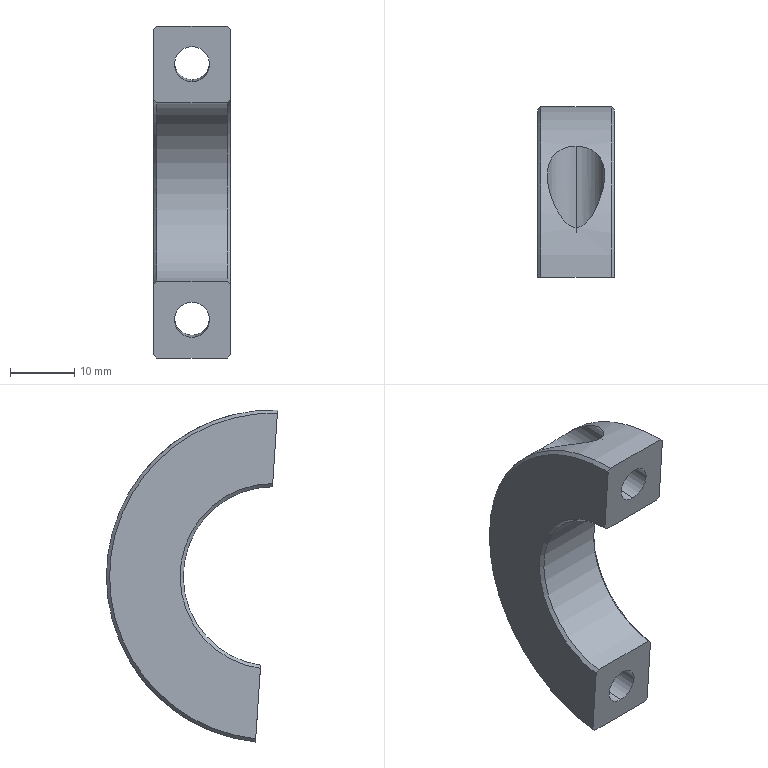Component | SolidWorks | TC020.05-07-1 | 1 solid | 20 faces | box 12 x 26.73 x 51.86 mm | volume 7193 mm3 | cylinder 10 | plane 6 | cone 4 | commonest cylinder face diameters 5.5 x4 9 x4 28 x1 52 x1 | material Q235A
build123d program:
from build123d import *

# Parameters (mm, degrees)
SKETCH1_W          = 12
SKETCH1_H          = 12
SKETCH2_W          = 52
SKETCH2_H          = 2
CUT_EXTRUDE1_DEPTH = 39.678
CHAMFER1_SIZE      = 0.5


with BuildPart() as part:
    # Sketch1 → Revolve1 (revolve)
    with BuildSketch(Plane.XY, mode=Mode.PRIVATE) as revolve1_sk:
        with Locations((0, 20)):
            Rectangle(SKETCH1_W, SKETCH1_H)
    revolve(revolve1_sk.sketch.rotate(Axis((0, 0, 0), (1, 0, 0)), 90), axis=Axis((0, 0, 0), (1, 0, 0)))

    # Sketch2 → Cut-Extrude1 (cut, through all)
    with BuildSketch(Plane(origin=(6, 0, 0), x_dir=(0, 0, -1), z_dir=(1, 0, 0))):
        Rectangle(SKETCH2_W, SKETCH2_H)
    extrude(amount=-CUT_EXTRUDE1_DEPTH, mode=Mode.SUBTRACT)


with BuildPart() as cut_extrude1_kept_piece:
    # of the separate pieces the step leaves, the one the design keeps (cut_extrude1_pieces_kept)
    add(part.part.solids().sort_by_distance((-6, 1, -13.964))[0])

    # Sketch5 → Cut-Revolve1 (revolve, cut)
    with BuildSketch(Plane(origin=(0, 0, 0), x_dir=(0, 0, -1), z_dir=(1, 0, 0))):
        Polygon((20, 31), (24.5, 31), (24.5, 6), (22.75, 6), (22.75, 1), (20, 1), align=None)
    cut_revolve1 = revolve(axis=Axis((0, -1.721, -20), (0, 1, 0)), mode=Mode.SUBTRACT)

    # Mirror1: Cut-Revolve1 across plane
    add(cut_revolve1.mirror(Plane.XY), mode=Mode.SUBTRACT)

    # Chamfer1
    chamfer1_edges = [cut_extrude1_kept_piece.edges().sort_by_distance(p)[0] for p in [
        (6, 26, 0),
        (-6, 26, 0),
        (-6, 14, 0),
        (6, 14, 0),
    ]]
    chamfer(chamfer1_edges, length=CHAMFER1_SIZE)


solid = cut_extrude1_kept_piece.part

# Placed as in the assembly
solid = solid.moved(Location((239.493, 30, 0), (3.804, -0.0003059, -0.0001204)))
STEP:
#1=COLOUR_RGB('',0.7922,0.8196,0.9333);
#2=FILL_AREA_STYLE_COLOUR('',#1);
#3=FILL_AREA_STYLE('',(#2));
#4=SURFACE_STYLE_FILL_AREA(#3);
#5=SURFACE_SIDE_STYLE('',(#4));
#6=SURFACE_STYLE_USAGE(.BOTH.,#5);
#7=PRESENTATION_STYLE_ASSIGNMENT((#6));
#8=CARTESIAN_POINT('',(9.429,1.357,0.9094));
#9=VERTEX_POINT('',#8);
#10=CARTESIAN_POINT('',(9.429,1.372,0.6933));
#11=VERTEX_POINT('',#10);
#12=CARTESIAN_POINT('',(9.429,1.365,0.8013));
#13=DIRECTION('',(0.,0.9978,0.06635));
#14=DIRECTION('',(0.,-0.06635,0.9978));
#15=AXIS2_PLACEMENT_3D('',#12,#13,#14);
#16=CIRCLE('',#15,0.1083);
#17=EDGE_CURVE('',#9,#11,#16,.T.);
#18=ORIENTED_EDGE('',*,*,#17,.T.);
#19=CARTESIAN_POINT('',(9.429,1.175,0.6802));
#20=VERTEX_POINT('',#19);
#21=CARTESIAN_POINT('',(9.429,1.068,0.6731));
#22=DIRECTION('',(0.,-0.9978,-0.06635));
#23=VECTOR('',#22,39.37);
#24=LINE('',#21,#23);
#25=EDGE_CURVE('',#11,#20,#24,.T.);
#26=ORIENTED_EDGE('',*,*,#25,.T.);
#27=CARTESIAN_POINT('',(9.429,1.161,0.8963));
#28=VERTEX_POINT('',#27);
#29=CARTESIAN_POINT('',(9.429,1.168,0.7883));
#30=DIRECTION('',(0.,0.9978,0.06635));
#31=DIRECTION('',(0.,-0.06635,0.9978));
#32=AXIS2_PLACEMENT_3D('',#29,#30,#31);
#33=CIRCLE('',#32,0.1083);
#34=EDGE_CURVE('',#28,#20,#33,.T.);
#35=ORIENTED_EDGE('',*,*,#34,.F.);
#36=CARTESIAN_POINT('',(9.429,1.054,0.8892));
#37=DIRECTION('',(0.,-0.9978,-0.06635));
#38=VECTOR('',#37,39.37);
#39=LINE('',#36,#38);
#40=EDGE_CURVE('',#9,#28,#39,.T.);
#41=ORIENTED_EDGE('',*,*,#40,.F.);
#42=EDGE_LOOP('',(#18,#26,#35,#41));
#43=FACE_OUTER_BOUND('',#42,.T.);
#44=CARTESIAN_POINT('',(9.429,1.061,0.7812));
#45=DIRECTION('',(0.,-0.9978,-0.06635));
#46=DIRECTION('',(0.,-0.06635,0.9978));
#47=AXIS2_PLACEMENT_3D('',#44,#45,#46);
#48=CYLINDRICAL_SURFACE('',#47,0.1083);
#49=ADVANCED_FACE('',(#43),#48,.F.);
#50=CARTESIAN_POINT('',(9.429,1.961,0.6634));
#51=VERTEX_POINT('',#50);
#52=CARTESIAN_POINT('',(9.429,1.459,0.9852));
#53=VERTEX_POINT('',#52);
#54=CARTESIAN_POINT('',(9.429,1.961,0.6634));
#55=CARTESIAN_POINT('',(9.445,1.961,0.6634));
#56=CARTESIAN_POINT('',(9.461,1.959,0.6655));
#57=CARTESIAN_POINT('',(9.491,1.952,0.6734));
#58=CARTESIAN_POINT('',(9.505,1.947,0.6791));
#59=CARTESIAN_POINT('',(9.531,1.934,0.6933));
#60=CARTESIAN_POINT('',(9.542,1.927,0.7015));
#61=CARTESIAN_POINT('',(9.557,1.914,0.7151));
#62=CARTESIAN_POINT('',(9.562,1.909,0.7198));
#63=CARTESIAN_POINT('',(9.57,1.899,0.7293));
#64=CARTESIAN_POINT('',(9.574,1.894,0.7342));
#65=CARTESIAN_POINT('',(9.581,1.884,0.7441));
#66=CARTESIAN_POINT('',(9.584,1.879,0.7491));
#67=CARTESIAN_POINT('',(9.589,1.868,0.7592));
#68=CARTESIAN_POINT('',(9.592,1.862,0.7643));
#69=CARTESIAN_POINT('',(9.598,1.845,0.7795));
#70=CARTESIAN_POINT('',(9.601,1.833,0.7894));
#71=CARTESIAN_POINT('',(9.605,1.808,0.809));
#72=CARTESIAN_POINT('',(9.606,1.796,0.8187));
#73=CARTESIAN_POINT('',(9.606,1.77,0.8374));
#74=CARTESIAN_POINT('',(9.605,1.757,0.8464));
#75=CARTESIAN_POINT('',(9.601,1.718,0.8723));
#76=CARTESIAN_POINT('',(9.595,1.691,0.8881));
#77=CARTESIAN_POINT('',(9.578,1.637,0.917));
#78=CARTESIAN_POINT('',(9.567,1.61,0.9299));
#79=CARTESIAN_POINT('',(9.548,1.57,0.9468));
#80=CARTESIAN_POINT('',(9.541,1.557,0.952));
#81=CARTESIAN_POINT('',(9.525,1.532,0.9618));
#82=CARTESIAN_POINT('',(9.516,1.519,0.9663));
#83=CARTESIAN_POINT('',(9.497,1.495,0.9743));
#84=CARTESIAN_POINT('',(9.486,1.484,0.9779));
#85=CARTESIAN_POINT('',(9.467,1.47,0.9819));
#86=CARTESIAN_POINT('',(9.46,1.466,0.9831));
#87=CARTESIAN_POINT('',(9.445,1.461,0.9847));
#88=CARTESIAN_POINT('',(9.437,1.459,0.9852));
#89=CARTESIAN_POINT('',(9.429,1.459,0.9852));
#90=B_SPLINE_CURVE_WITH_KNOTS('',3,(#54,#55,#56,#57,#58,#59,#60,#61,#62,#63,#64,#65,#66,#67,#68,#69,#70,#71,#72,#73,#74,#75,#76,#77,#78,#79,#80,#81,#82,#83,#84,#85,#86,#87,#88,#89),.UNSPECIFIED.,.F.,.F.,(4,2,2,2,2,2,2,2,2,2,2,2,2,2,2,2,2,4),(0.0194,0.02061,0.02182,0.02303,0.02364,0.02424,0.02485,0.02546,0.02667,0.02788,0.02909,0.03152,0.03394,0.03515,0.03637,0.03758,0.03818,0.03879),.UNSPECIFIED.);
#91=EDGE_CURVE('',#51,#53,#90,.T.);
#92=ORIENTED_EDGE('',*,*,#91,.F.);
#93=CARTESIAN_POINT('',(9.429,1.376,0.6246));
#94=VERTEX_POINT('',#93);
#95=CARTESIAN_POINT('',(9.429,1.073,0.6044));
#96=DIRECTION('',(0.,-0.9978,-0.06635));
#97=VECTOR('',#96,39.37);
#98=LINE('',#95,#97);
#99=EDGE_CURVE('',#51,#94,#98,.T.);
#100=ORIENTED_EDGE('',*,*,#99,.T.);
#101=CARTESIAN_POINT('',(9.429,1.353,0.9781));
#102=VERTEX_POINT('',#101);
#103=CARTESIAN_POINT('',(9.429,1.365,0.8013));
#104=DIRECTION('',(0.,0.9978,0.06635));
#105=DIRECTION('',(0.,-0.06635,0.9978));
#106=AXIS2_PLACEMENT_3D('',#103,#104,#105);
#107=CIRCLE('',#106,0.1772);
#108=EDGE_CURVE('',#102,#94,#107,.T.);
#109=ORIENTED_EDGE('',*,*,#108,.F.);
#110=CARTESIAN_POINT('',(9.429,1.049,0.9579));
#111=DIRECTION('',(0.,-0.9978,-0.06635));
#112=VECTOR('',#111,39.37);
#113=LINE('',#110,#112);
#114=EDGE_CURVE('',#53,#102,#113,.T.);
#115=ORIENTED_EDGE('',*,*,#114,.F.);
#116=EDGE_LOOP('',(#92,#100,#109,#115));
#117=FACE_OUTER_BOUND('',#116,.T.);
#118=CARTESIAN_POINT('',(9.429,1.061,0.7812));
#119=DIRECTION('',(0.,-0.9978,-0.06635));
#120=DIRECTION('',(0.,-0.06635,0.9978));
#121=AXIS2_PLACEMENT_3D('',#118,#119,#120);
#122=CYLINDRICAL_SURFACE('',#121,0.1772);
#123=ADVANCED_FACE('',(#117),#122,.F.);
#124=CARTESIAN_POINT('',(9.429,1.462,-0.662));
#125=VERTEX_POINT('',#124);
#126=CARTESIAN_POINT('',(9.429,1.476,-0.878));
#127=VERTEX_POINT('',#126);
#128=CARTESIAN_POINT('',(9.429,1.469,-0.77));
#129=DIRECTION('',(0.,-0.9978,-0.06635));
#130=DIRECTION('',(0.,0.06635,-0.9978));
#131=AXIS2_PLACEMENT_3D('',#128,#129,#130);
#132=CIRCLE('',#131,0.1083);
#133=EDGE_CURVE('',#125,#127,#132,.T.);
#134=ORIENTED_EDGE('',*,*,#133,.F.);
#135=CARTESIAN_POINT('',(9.429,1.265,-0.675));
#136=VERTEX_POINT('',#135);
#137=CARTESIAN_POINT('',(9.429,1.159,-0.6821));
#138=DIRECTION('',(0.,-0.9978,-0.06635));
#139=VECTOR('',#138,39.37);
#140=LINE('',#137,#139);
#141=EDGE_CURVE('',#125,#136,#140,.T.);
#142=ORIENTED_EDGE('',*,*,#141,.T.);
#143=CARTESIAN_POINT('',(9.429,1.28,-0.8911));
#144=VERTEX_POINT('',#143);
#145=CARTESIAN_POINT('',(9.429,1.273,-0.7831));
#146=DIRECTION('',(0.,-0.9978,-0.06635));
#147=DIRECTION('',(0.,0.06635,-0.9978));
#148=AXIS2_PLACEMENT_3D('',#145,#146,#147);
#149=CIRCLE('',#148,0.1083);
#150=EDGE_CURVE('',#136,#144,#149,.T.);
#151=ORIENTED_EDGE('',*,*,#150,.T.);
#152=CARTESIAN_POINT('',(9.429,1.173,-0.8982));
#153=DIRECTION('',(0.,-0.9978,-0.06635));
#154=VECTOR('',#153,39.37);
#155=LINE('',#152,#154);
#156=EDGE_CURVE('',#127,#144,#155,.T.);
#157=ORIENTED_EDGE('',*,*,#156,.F.);
#158=EDGE_LOOP('',(#134,#142,#151,#157));
#159=FACE_OUTER_BOUND('',#158,.T.);
#160=CARTESIAN_POINT('',(9.429,1.166,-0.7902));
#161=DIRECTION('',(0.,-0.9978,-0.06635));
#162=DIRECTION('',(0.,0.06635,-0.9978));
#163=AXIS2_PLACEMENT_3D('',#160,#161,#162);
#164=CYLINDRICAL_SURFACE('',#163,0.1083);
#165=ADVANCED_FACE('',(#159),#164,.F.);
#166=CARTESIAN_POINT('',(9.429,2.042,-0.5544));
#167=VERTEX_POINT('',#166);
#168=CARTESIAN_POINT('',(9.429,1.587,-0.9397));
#169=VERTEX_POINT('',#168);
#170=CARTESIAN_POINT('',(9.429,2.042,-0.5544));
#171=CARTESIAN_POINT('',(9.413,2.042,-0.5544));
#172=CARTESIAN_POINT('',(9.397,2.04,-0.5566));
#173=CARTESIAN_POINT('',(9.367,2.034,-0.5654));
#174=CARTESIAN_POINT('',(9.353,2.03,-0.5717));
#175=CARTESIAN_POINT('',(9.327,2.019,-0.5875));
#176=CARTESIAN_POINT('',(9.316,2.013,-0.5966));
#177=CARTESIAN_POINT('',(9.301,2.002,-0.6118));
#178=CARTESIAN_POINT('',(9.296,1.998,-0.6171));
#179=CARTESIAN_POINT('',(9.288,1.99,-0.6278));
#180=CARTESIAN_POINT('',(9.284,1.985,-0.6333));
#181=CARTESIAN_POINT('',(9.277,1.976,-0.6445));
#182=CARTESIAN_POINT('',(9.274,1.972,-0.6501));
#183=CARTESIAN_POINT('',(9.268,1.962,-0.6616));
#184=CARTESIAN_POINT('',(9.266,1.957,-0.6674));
#185=CARTESIAN_POINT('',(9.26,1.942,-0.6847));
#186=CARTESIAN_POINT('',(9.257,1.932,-0.6962));
#187=CARTESIAN_POINT('',(9.253,1.91,-0.7188));
#188=CARTESIAN_POINT('',(9.252,1.899,-0.7301));
#189=CARTESIAN_POINT('',(9.252,1.876,-0.7521));
#190=CARTESIAN_POINT('',(9.252,1.864,-0.7627));
#191=CARTESIAN_POINT('',(9.257,1.828,-0.7935));
#192=CARTESIAN_POINT('',(9.263,1.804,-0.8127));
#193=CARTESIAN_POINT('',(9.28,1.754,-0.8486));
#194=CARTESIAN_POINT('',(9.29,1.729,-0.8649));
#195=CARTESIAN_POINT('',(9.31,1.692,-0.8869));
#196=CARTESIAN_POINT('',(9.317,1.68,-0.8938));
#197=CARTESIAN_POINT('',(9.333,1.656,-0.9069));
#198=CARTESIAN_POINT('',(9.341,1.644,-0.9131));
#199=CARTESIAN_POINT('',(9.361,1.621,-0.9242));
#200=CARTESIAN_POINT('',(9.372,1.611,-0.9292));
#201=CARTESIAN_POINT('',(9.391,1.598,-0.935));
#202=CARTESIAN_POINT('',(9.398,1.594,-0.9367));
#203=CARTESIAN_POINT('',(9.413,1.589,-0.939));
#204=CARTESIAN_POINT('',(9.421,1.587,-0.9397));
#205=CARTESIAN_POINT('',(9.429,1.587,-0.9397));
#206=B_SPLINE_CURVE_WITH_KNOTS('',3,(#170,#171,#172,#173,#174,#175,#176,#177,#178,#179,#180,#181,#182,#183,#184,#185,#186,#187,#188,#189,#190,#191,#192,#193,#194,#195,#196,#197,#198,#199,#200,#201,#202,#203,#204,#205),.UNSPECIFIED.,.F.,.F.,(4,2,2,2,2,2,2,2,2,2,2,2,2,2,2,2,2,4),(0.0194,0.02061,0.02182,0.02303,0.02364,0.02424,0.02485,0.02546,0.02667,0.02788,0.02909,0.03152,0.03394,0.03515,0.03637,0.03758,0.03818,0.03879),.UNSPECIFIED.);
#207=EDGE_CURVE('',#167,#169,#206,.T.);
#208=ORIENTED_EDGE('',*,*,#207,.F.);
#209=CARTESIAN_POINT('',(9.429,1.457,-0.5932));
#210=VERTEX_POINT('',#209);
#211=CARTESIAN_POINT('',(9.429,1.154,-0.6134));
#212=DIRECTION('',(0.,-0.9978,-0.06635));
#213=VECTOR('',#212,39.37);
#214=LINE('',#211,#213);
#215=EDGE_CURVE('',#167,#210,#214,.T.);
#216=ORIENTED_EDGE('',*,*,#215,.T.);
#217=CARTESIAN_POINT('',(9.429,1.481,-0.9468));
#218=VERTEX_POINT('',#217);
#219=CARTESIAN_POINT('',(9.429,1.469,-0.77));
#220=DIRECTION('',(0.,-0.9978,-0.06635));
#221=DIRECTION('',(0.,0.06635,-0.9978));
#222=AXIS2_PLACEMENT_3D('',#219,#220,#221);
#223=CIRCLE('',#222,0.1772);
#224=EDGE_CURVE('',#210,#218,#223,.T.);
#225=ORIENTED_EDGE('',*,*,#224,.T.);
#226=CARTESIAN_POINT('',(9.429,1.177,-0.9669));
#227=DIRECTION('',(0.,-0.9978,-0.06635));
#228=VECTOR('',#227,39.37);
#229=LINE('',#226,#228);
#230=EDGE_CURVE('',#169,#218,#229,.T.);
#231=ORIENTED_EDGE('',*,*,#230,.F.);
#232=EDGE_LOOP('',(#208,#216,#225,#231));
#233=FACE_OUTER_BOUND('',#232,.T.);
#234=CARTESIAN_POINT('',(9.429,1.166,-0.7902));
#235=DIRECTION('',(0.,-0.9978,-0.06635));
#236=DIRECTION('',(0.,0.06635,-0.9978));
#237=AXIS2_PLACEMENT_3D('',#234,#235,#236);
#238=CYLINDRICAL_SURFACE('',#237,0.1772);
#239=ADVANCED_FACE('',(#233),#238,.F.);
#240=CARTESIAN_POINT('',(9.645,1.184,0.5512));
#241=VERTEX_POINT('',#240);
#242=CARTESIAN_POINT('',(9.212,1.184,0.5512));
#243=VERTEX_POINT('',#242);
#244=CARTESIAN_POINT('',(9.429,1.184,0.5512));
#245=DIRECTION('',(-1.,0.,0.));
#246=VECTOR('',#245,39.37);
#247=LINE('',#244,#246);
#248=EDGE_CURVE('',#241,#243,#247,.T.);
#249=ORIENTED_EDGE('',*,*,#248,.T.);
#250=CARTESIAN_POINT('',(9.212,1.257,-0.5459));
#251=VERTEX_POINT('',#250);
#252=CARTESIAN_POINT('',(9.212,1.181,0.));
#253=DIRECTION('',(-1.,0.,0.));
#254=DIRECTION('',(0.,0.06635,-0.9978));
#255=AXIS2_PLACEMENT_3D('',#252,#253,#254);
#256=CIRCLE('',#255,0.5512);
#257=EDGE_CURVE('',#243,#251,#256,.T.);
#258=ORIENTED_EDGE('',*,*,#257,.T.);
#259=CARTESIAN_POINT('',(9.645,1.257,-0.5459));
#260=VERTEX_POINT('',#259);
#261=CARTESIAN_POINT('',(9.429,1.257,-0.5459));
#262=DIRECTION('',(1.,0.,0.));
#263=VECTOR('',#262,39.37);
#264=LINE('',#261,#263);
#265=EDGE_CURVE('',#251,#260,#264,.T.);
#266=ORIENTED_EDGE('',*,*,#265,.T.);
#267=CARTESIAN_POINT('',(9.645,1.181,0.));
#268=DIRECTION('',(1.,0.,0.));
#269=DIRECTION('',(0.,-0.06635,0.9978));
#270=AXIS2_PLACEMENT_3D('',#267,#268,#269);
#271=CIRCLE('',#270,0.5512);
#272=EDGE_CURVE('',#260,#241,#271,.T.);
#273=ORIENTED_EDGE('',*,*,#272,.T.);
#274=EDGE_LOOP('',(#249,#258,#266,#273));
#275=FACE_OUTER_BOUND('',#274,.T.);
#276=CARTESIAN_POINT('',(9.429,1.181,0.));
#277=DIRECTION('',(-1.,0.,0.));
#278=DIRECTION('',(0.,-0.06635,0.9978));
#279=AXIS2_PLACEMENT_3D('',#276,#277,#278);
#280=CYLINDRICAL_SURFACE('',#279,0.5512);
#281=ADVANCED_FACE('',(#275),#280,.F.);
#282=CARTESIAN_POINT('',(9.665,1.183,0.5709));
#283=VERTEX_POINT('',#282);
#284=CARTESIAN_POINT('',(9.665,1.154,1.004));
#285=VERTEX_POINT('',#284);
#286=CARTESIAN_POINT('',(9.665,1.152,1.024));
#287=DIRECTION('',(0.,-0.06635,0.9978));
#288=VECTOR('',#287,39.37);
#289=LINE('',#286,#288);
#290=EDGE_CURVE('',#283,#285,#289,.T.);
#291=ORIENTED_EDGE('',*,*,#290,.F.);
#292=CARTESIAN_POINT('',(9.665,1.258,-0.5656));
#293=VERTEX_POINT('',#292);
#294=CARTESIAN_POINT('',(9.665,1.181,0.));
#295=DIRECTION('',(-1.,0.,0.));
#296=DIRECTION('',(0.,-0.06635,0.9978));
#297=AXIS2_PLACEMENT_3D('',#294,#295,#296);
#298=CIRCLE('',#297,0.5709);
#299=EDGE_CURVE('',#283,#293,#298,.T.);
#300=ORIENTED_EDGE('',*,*,#299,.T.);
#301=CARTESIAN_POINT('',(9.665,1.287,-0.9983));
#302=VERTEX_POINT('',#301);
#303=CARTESIAN_POINT('',(9.665,1.152,1.024));
#304=DIRECTION('',(0.,-0.06635,0.9978));
#305=VECTOR('',#304,39.37);
#306=LINE('',#303,#305);
#307=EDGE_CURVE('',#302,#293,#306,.T.);
#308=ORIENTED_EDGE('',*,*,#307,.F.);
#309=CARTESIAN_POINT('',(9.665,1.181,0.));
#310=DIRECTION('',(1.,0.,0.));
#311=DIRECTION('',(0.,-0.06635,0.9978));
#312=AXIS2_PLACEMENT_3D('',#309,#310,#311);
#313=CIRCLE('',#312,1.004);
#314=EDGE_CURVE('',#302,#285,#313,.T.);
#315=ORIENTED_EDGE('',*,*,#314,.T.);
#316=EDGE_LOOP('',(#291,#300,#308,#315));
#317=FACE_OUTER_BOUND('',#316,.T.);
#318=CARTESIAN_POINT('',(9.665,1.731,0.03657));
#319=DIRECTION('',(-1.,0.,0.));
#320=DIRECTION('',(0.,-0.06635,0.9978));
#321=AXIS2_PLACEMENT_3D('',#318,#319,#320);
#322=PLANE('',#321);
#323=ADVANCED_FACE('',(#317),#322,.F.);
#324=CARTESIAN_POINT('',(9.429,1.459,0.9852));
#325=CARTESIAN_POINT('',(9.421,1.459,0.9852));
#326=CARTESIAN_POINT('',(9.413,1.461,0.9847));
#327=CARTESIAN_POINT('',(9.398,1.466,0.9831));
#328=CARTESIAN_POINT('',(9.391,1.47,0.982));
#329=CARTESIAN_POINT('',(9.378,1.479,0.9792));
#330=CARTESIAN_POINT('',(9.372,1.484,0.9777));
#331=CARTESIAN_POINT('',(9.361,1.495,0.9742));
#332=CARTESIAN_POINT('',(9.356,1.501,0.9724));
#333=CARTESIAN_POINT('',(9.341,1.519,0.9664));
#334=CARTESIAN_POINT('',(9.333,1.532,0.9618));
#335=CARTESIAN_POINT('',(9.317,1.557,0.9521));
#336=CARTESIAN_POINT('',(9.31,1.57,0.9468));
#337=CARTESIAN_POINT('',(9.297,1.597,0.9355));
#338=CARTESIAN_POINT('',(9.291,1.61,0.9295));
#339=CARTESIAN_POINT('',(9.28,1.637,0.9165));
#340=CARTESIAN_POINT('',(9.275,1.651,0.9097));
#341=CARTESIAN_POINT('',(9.263,1.691,0.8881));
#342=CARTESIAN_POINT('',(9.257,1.718,0.8723));
#343=CARTESIAN_POINT('',(9.252,1.757,0.8463));
#344=CARTESIAN_POINT('',(9.252,1.77,0.8372));
#345=CARTESIAN_POINT('',(9.252,1.796,0.8185));
#346=CARTESIAN_POINT('',(9.253,1.809,0.8089));
#347=CARTESIAN_POINT('',(9.257,1.833,0.7893));
#348=CARTESIAN_POINT('',(9.26,1.845,0.7792));
#349=CARTESIAN_POINT('',(9.268,1.868,0.759));
#350=CARTESIAN_POINT('',(9.274,1.879,0.7489));
#351=CARTESIAN_POINT('',(9.287,1.9,0.7291));
#352=CARTESIAN_POINT('',(9.296,1.909,0.7194));
#353=CARTESIAN_POINT('',(9.311,1.922,0.7059));
#354=CARTESIAN_POINT('',(9.316,1.926,0.7016));
#355=CARTESIAN_POINT('',(9.327,1.934,0.6935));
#356=CARTESIAN_POINT('',(9.334,1.938,0.6896));
#357=CARTESIAN_POINT('',(9.346,1.944,0.6826));
#358=CARTESIAN_POINT('',(9.353,1.947,0.6794));
#359=CARTESIAN_POINT('',(9.367,1.952,0.6738));
#360=CARTESIAN_POINT('',(9.374,1.954,0.6714));
#361=CARTESIAN_POINT('',(9.397,1.959,0.6655));
#362=CARTESIAN_POINT('',(9.413,1.961,0.6634));
#363=CARTESIAN_POINT('',(9.429,1.961,0.6634));
#364=B_SPLINE_CURVE_WITH_KNOTS('',3,(#324,#325,#326,#327,#328,#329,#330,#331,#332,#333,#334,#335,#336,#337,#338,#339,#340,#341,#342,#343,#344,#345,#346,#347,#348,#349,#350,#351,#352,#353,#354,#355,#356,#357,#358,#359,#360,#361,#362,#363),.UNSPECIFIED.,.F.,.F.,(4,2,2,2,2,2,2,2,2,2,2,2,2,2,2,2,2,2,2,4),(0.,0.0006061,0.001212,0.001818,0.002424,0.003637,0.004849,0.006061,0.007273,0.009698,0.01091,0.01212,0.01333,0.01455,0.01576,0.01637,0.01697,0.01758,0.01818,0.0194),.UNSPECIFIED.);
#365=EDGE_CURVE('',#53,#51,#364,.T.);
#366=ORIENTED_EDGE('',*,*,#365,.T.);
#367=ORIENTED_EDGE('',*,*,#91,.T.);
#368=EDGE_LOOP('',(#366,#367));
#369=FACE_BOUND('',#368,.T.);
#370=CARTESIAN_POINT('',(9.429,1.587,-0.9397));
#371=CARTESIAN_POINT('',(9.437,1.587,-0.9397));
#372=CARTESIAN_POINT('',(9.445,1.589,-0.9391));
#373=CARTESIAN_POINT('',(9.46,1.594,-0.9367));
#374=CARTESIAN_POINT('',(9.467,1.598,-0.935));
#375=CARTESIAN_POINT('',(9.479,1.606,-0.9311));
#376=CARTESIAN_POINT('',(9.485,1.611,-0.9289));
#377=CARTESIAN_POINT('',(9.497,1.622,-0.924));
#378=CARTESIAN_POINT('',(9.502,1.627,-0.9214));
#379=CARTESIAN_POINT('',(9.516,1.644,-0.9131));
#380=CARTESIAN_POINT('',(9.525,1.656,-0.907));
#381=CARTESIAN_POINT('',(9.541,1.68,-0.8939));
#382=CARTESIAN_POINT('',(9.548,1.692,-0.887));
#383=CARTESIAN_POINT('',(9.561,1.717,-0.8722));
#384=CARTESIAN_POINT('',(9.567,1.729,-0.8645));
#385=CARTESIAN_POINT('',(9.577,1.755,-0.8481));
#386=CARTESIAN_POINT('',(9.582,1.767,-0.8395));
#387=CARTESIAN_POINT('',(9.595,1.804,-0.8127));
#388=CARTESIAN_POINT('',(9.601,1.828,-0.7936));
#389=CARTESIAN_POINT('',(9.605,1.864,-0.7625));
#390=CARTESIAN_POINT('',(9.606,1.876,-0.7518));
#391=CARTESIAN_POINT('',(9.606,1.899,-0.7299));
#392=CARTESIAN_POINT('',(9.605,1.91,-0.7188));
#393=CARTESIAN_POINT('',(9.601,1.932,-0.6961));
#394=CARTESIAN_POINT('',(9.598,1.942,-0.6844));
#395=CARTESIAN_POINT('',(9.589,1.963,-0.6613));
#396=CARTESIAN_POINT('',(9.584,1.972,-0.6499));
#397=CARTESIAN_POINT('',(9.57,1.99,-0.6276));
#398=CARTESIAN_POINT('',(9.562,1.998,-0.6166));
#399=CARTESIAN_POINT('',(9.547,2.009,-0.6016));
#400=CARTESIAN_POINT('',(9.542,2.013,-0.5968));
#401=CARTESIAN_POINT('',(9.53,2.019,-0.5877));
#402=CARTESIAN_POINT('',(9.524,2.022,-0.5834));
#403=CARTESIAN_POINT('',(9.511,2.028,-0.5756));
#404=CARTESIAN_POINT('',(9.505,2.03,-0.572));
#405=CARTESIAN_POINT('',(9.491,2.034,-0.5658));
#406=CARTESIAN_POINT('',(9.483,2.036,-0.5631));
#407=CARTESIAN_POINT('',(9.461,2.04,-0.5566));
#408=CARTESIAN_POINT('',(9.445,2.042,-0.5544));
#409=CARTESIAN_POINT('',(9.429,2.042,-0.5544));
#410=B_SPLINE_CURVE_WITH_KNOTS('',3,(#370,#371,#372,#373,#374,#375,#376,#377,#378,#379,#380,#381,#382,#383,#384,#385,#386,#387,#388,#389,#390,#391,#392,#393,#394,#395,#396,#397,#398,#399,#400,#401,#402,#403,#404,#405,#406,#407,#408,#409),.UNSPECIFIED.,.F.,.F.,(4,2,2,2,2,2,2,2,2,2,2,2,2,2,2,2,2,2,2,4),(0.,0.0006061,0.001212,0.001818,0.002424,0.003637,0.004849,0.006061,0.007273,0.009698,0.01091,0.01212,0.01333,0.01455,0.01576,0.01637,0.01697,0.01758,0.01818,0.0194),.UNSPECIFIED.);
#411=EDGE_CURVE('',#169,#167,#410,.T.);
#412=ORIENTED_EDGE('',*,*,#411,.T.);
#413=ORIENTED_EDGE('',*,*,#207,.T.);
#414=EDGE_LOOP('',(#412,#413));
#415=FACE_BOUND('',#414,.T.);
#416=CARTESIAN_POINT('',(9.645,1.288,-1.018));
#417=VERTEX_POINT('',#416);
#418=CARTESIAN_POINT('',(9.212,1.288,-1.018));
#419=VERTEX_POINT('',#418);
#420=CARTESIAN_POINT('',(9.429,1.288,-1.018));
#421=DIRECTION('',(-1.,0.,0.));
#422=VECTOR('',#421,39.37);
#423=LINE('',#420,#422);
#424=EDGE_CURVE('',#417,#419,#423,.T.);
#425=ORIENTED_EDGE('',*,*,#424,.T.);
#426=CARTESIAN_POINT('',(9.212,1.153,1.023));
#427=VERTEX_POINT('',#426);
#428=CARTESIAN_POINT('',(9.212,1.181,0.));
#429=DIRECTION('',(1.,0.,0.));
#430=DIRECTION('',(0.,0.06635,-0.9978));
#431=AXIS2_PLACEMENT_3D('',#428,#429,#430);
#432=CIRCLE('',#431,1.024);
#433=EDGE_CURVE('',#419,#427,#432,.T.);
#434=ORIENTED_EDGE('',*,*,#433,.T.);
#435=CARTESIAN_POINT('',(9.645,1.153,1.023));
#436=VERTEX_POINT('',#435);
#437=CARTESIAN_POINT('',(9.429,1.153,1.023));
#438=DIRECTION('',(1.,0.,0.));
#439=VECTOR('',#438,39.37);
#440=LINE('',#437,#439);
#441=EDGE_CURVE('',#427,#436,#440,.T.);
#442=ORIENTED_EDGE('',*,*,#441,.T.);
#443=CARTESIAN_POINT('',(9.645,1.181,0.));
#444=DIRECTION('',(-1.,0.,0.));
#445=DIRECTION('',(0.,-0.06635,0.9978));
#446=AXIS2_PLACEMENT_3D('',#443,#444,#445);
#447=CIRCLE('',#446,1.024);
#448=EDGE_CURVE('',#436,#417,#447,.T.);
#449=ORIENTED_EDGE('',*,*,#448,.T.);
#450=EDGE_LOOP('',(#425,#434,#442,#449));
#451=FACE_OUTER_BOUND('',#450,.T.);
#452=CARTESIAN_POINT('',(9.429,1.181,0.));
#453=DIRECTION('',(-1.,0.,0.));
#454=DIRECTION('',(0.,-0.06635,0.9978));
#455=AXIS2_PLACEMENT_3D('',#452,#453,#454);
#456=CYLINDRICAL_SURFACE('',#455,1.024);
#457=ADVANCED_FACE('',(#369,#415,#451),#456,.T.);
#458=CARTESIAN_POINT('',(9.193,1.287,-0.9983));
#459=VERTEX_POINT('',#458);
#460=CARTESIAN_POINT('',(9.193,1.258,-0.5656));
#461=VERTEX_POINT('',#460);
#462=CARTESIAN_POINT('',(9.193,1.152,1.024));
#463=DIRECTION('',(0.,-0.06635,0.9978));
#464=VECTOR('',#463,39.37);
#465=LINE('',#462,#464);
#466=EDGE_CURVE('',#459,#461,#465,.T.);
#467=ORIENTED_EDGE('',*,*,#466,.T.);
#468=CARTESIAN_POINT('',(9.193,1.183,0.5709));
#469=VERTEX_POINT('',#468);
#470=CARTESIAN_POINT('',(9.193,1.181,0.));
#471=DIRECTION('',(1.,0.,0.));
#472=DIRECTION('',(0.,0.06635,-0.9978));
#473=AXIS2_PLACEMENT_3D('',#470,#471,#472);
#474=CIRCLE('',#473,0.5709);
#475=EDGE_CURVE('',#461,#469,#474,.T.);
#476=ORIENTED_EDGE('',*,*,#475,.T.);
#477=CARTESIAN_POINT('',(9.193,1.154,1.004));
#478=VERTEX_POINT('',#477);
#479=CARTESIAN_POINT('',(9.193,1.152,1.024));
#480=DIRECTION('',(0.,-0.06635,0.9978));
#481=VECTOR('',#480,39.37);
#482=LINE('',#479,#481);
#483=EDGE_CURVE('',#469,#478,#482,.T.);
#484=ORIENTED_EDGE('',*,*,#483,.T.);
#485=CARTESIAN_POINT('',(9.193,1.181,0.));
#486=DIRECTION('',(-1.,0.,0.));
#487=DIRECTION('',(0.,0.06635,-0.9978));
#488=AXIS2_PLACEMENT_3D('',#485,#486,#487);
#489=CIRCLE('',#488,1.004);
#490=EDGE_CURVE('',#478,#459,#489,.T.);
#491=ORIENTED_EDGE('',*,*,#490,.T.);
#492=EDGE_LOOP('',(#467,#476,#484,#491));
#493=FACE_OUTER_BOUND('',#492,.T.);
#494=CARTESIAN_POINT('',(9.193,1.731,0.03657));
#495=DIRECTION('',(1.,0.,0.));
#496=DIRECTION('',(0.,0.06635,-0.9978));
#497=AXIS2_PLACEMENT_3D('',#494,#495,#496);
#498=PLANE('',#497);
#499=ADVANCED_FACE('',(#493),#498,.F.);
#500=ORIENTED_EDGE('',*,*,#34,.T.);
#501=CARTESIAN_POINT('',(9.429,1.168,0.7883));
#502=DIRECTION('',(0.,0.9978,0.06635));
#503=DIRECTION('',(0.,-0.06635,0.9978));
#504=AXIS2_PLACEMENT_3D('',#501,#502,#503);
#505=CIRCLE('',#504,0.1083);
#506=EDGE_CURVE('',#20,#28,#505,.T.);
#507=ORIENTED_EDGE('',*,*,#506,.T.);
#508=EDGE_LOOP('',(#500,#507));
#509=FACE_BOUND('',#508,.T.);
#510=ORIENTED_EDGE('',*,*,#483,.F.);
#511=CARTESIAN_POINT('',(9.193,1.183,0.5709));
#512=CARTESIAN_POINT('',(9.199,1.183,0.5643));
#513=CARTESIAN_POINT('',(9.206,1.183,0.5577));
#514=CARTESIAN_POINT('',(9.212,1.184,0.5512));
#515=B_SPLINE_CURVE_WITH_KNOTS('',3,(#511,#512,#513,#514),.UNSPECIFIED.,.F.,.F.,(4,4),(0.,0.000708),.UNSPECIFIED.);
#516=EDGE_CURVE('',#469,#243,#515,.T.);
#517=ORIENTED_EDGE('',*,*,#516,.T.);
#518=ORIENTED_EDGE('',*,*,#248,.F.);
#519=CARTESIAN_POINT('',(9.645,1.184,0.5512));
#520=CARTESIAN_POINT('',(9.652,1.183,0.5577));
#521=CARTESIAN_POINT('',(9.659,1.183,0.5643));
#522=CARTESIAN_POINT('',(9.665,1.183,0.5709));
#523=B_SPLINE_CURVE_WITH_KNOTS('',3,(#519,#520,#521,#522),.UNSPECIFIED.,.F.,.F.,(4,4),(0.,0.000708),.UNSPECIFIED.);
#524=EDGE_CURVE('',#241,#283,#523,.T.);
#525=ORIENTED_EDGE('',*,*,#524,.T.);
#526=ORIENTED_EDGE('',*,*,#290,.T.);
#527=CARTESIAN_POINT('',(9.665,1.154,1.004));
#528=CARTESIAN_POINT('',(9.659,1.153,1.01));
#529=CARTESIAN_POINT('',(9.652,1.153,1.017));
#530=CARTESIAN_POINT('',(9.645,1.153,1.023));
#531=B_SPLINE_CURVE_WITH_KNOTS('',3,(#527,#528,#529,#530),.UNSPECIFIED.,.F.,.F.,(4,4),(0.,0.0007074),.UNSPECIFIED.);
#532=EDGE_CURVE('',#285,#436,#531,.T.);
#533=ORIENTED_EDGE('',*,*,#532,.T.);
#534=ORIENTED_EDGE('',*,*,#441,.F.);
#535=CARTESIAN_POINT('',(9.212,1.153,1.023));
#536=CARTESIAN_POINT('',(9.206,1.153,1.017));
#537=CARTESIAN_POINT('',(9.199,1.153,1.01));
#538=CARTESIAN_POINT('',(9.193,1.154,1.004));
#539=B_SPLINE_CURVE_WITH_KNOTS('',3,(#535,#536,#537,#538),.UNSPECIFIED.,.F.,.F.,(4,4),(0.,0.0007074),.UNSPECIFIED.);
#540=EDGE_CURVE('',#427,#478,#539,.T.);
#541=ORIENTED_EDGE('',*,*,#540,.T.);
#542=EDGE_LOOP('',(#510,#517,#518,#525,#526,#533,#534,#541));
#543=FACE_OUTER_BOUND('',#542,.T.);
#544=CARTESIAN_POINT('',(9.193,1.152,1.024));
#545=DIRECTION('',(0.,0.9978,0.06635));
#546=DIRECTION('',(0.,-0.06635,0.9978));
#547=AXIS2_PLACEMENT_3D('',#544,#545,#546);
#548=PLANE('',#547);
#549=ADVANCED_FACE('',(#509,#543),#548,.F.);
#550=CARTESIAN_POINT('',(9.429,1.273,-0.7831));
#551=DIRECTION('',(0.,-0.9978,-0.06635));
#552=DIRECTION('',(0.,0.06635,-0.9978));
#553=AXIS2_PLACEMENT_3D('',#550,#551,#552);
#554=CIRCLE('',#553,0.1083);
#555=EDGE_CURVE('',#144,#136,#554,.T.);
#556=ORIENTED_EDGE('',*,*,#555,.F.);
#557=ORIENTED_EDGE('',*,*,#150,.F.);
#558=EDGE_LOOP('',(#556,#557));
#559=FACE_BOUND('',#558,.T.);
#560=ORIENTED_EDGE('',*,*,#265,.F.);
#561=CARTESIAN_POINT('',(9.212,1.257,-0.5459));
#562=CARTESIAN_POINT('',(9.206,1.257,-0.5525));
#563=CARTESIAN_POINT('',(9.199,1.258,-0.5591));
#564=CARTESIAN_POINT('',(9.193,1.258,-0.5656));
#565=B_SPLINE_CURVE_WITH_KNOTS('',3,(#561,#562,#563,#564),.UNSPECIFIED.,.F.,.F.,(4,4),(0.,0.000708),.UNSPECIFIED.);
#566=EDGE_CURVE('',#251,#461,#565,.T.);
#567=ORIENTED_EDGE('',*,*,#566,.T.);
#568=ORIENTED_EDGE('',*,*,#466,.F.);
#569=CARTESIAN_POINT('',(9.193,1.287,-0.9983));
#570=CARTESIAN_POINT('',(9.199,1.287,-1.005));
#571=CARTESIAN_POINT('',(9.206,1.288,-1.011));
#572=CARTESIAN_POINT('',(9.212,1.288,-1.018));
#573=B_SPLINE_CURVE_WITH_KNOTS('',3,(#569,#570,#571,#572),.UNSPECIFIED.,.F.,.F.,(4,4),(0.,0.0007074),.UNSPECIFIED.);
#574=EDGE_CURVE('',#459,#419,#573,.T.);
#575=ORIENTED_EDGE('',*,*,#574,.T.);
#576=ORIENTED_EDGE('',*,*,#424,.F.);
#577=CARTESIAN_POINT('',(9.645,1.288,-1.018));
#578=CARTESIAN_POINT('',(9.652,1.288,-1.011));
#579=CARTESIAN_POINT('',(9.659,1.287,-1.005));
#580=CARTESIAN_POINT('',(9.665,1.287,-0.9983));
#581=B_SPLINE_CURVE_WITH_KNOTS('',3,(#577,#578,#579,#580),.UNSPECIFIED.,.F.,.F.,(4,4),(0.,0.0007074),.UNSPECIFIED.);
#582=EDGE_CURVE('',#417,#302,#581,.T.);
#583=ORIENTED_EDGE('',*,*,#582,.T.);
#584=ORIENTED_EDGE('',*,*,#307,.T.);
#585=CARTESIAN_POINT('',(9.665,1.258,-0.5656));
#586=CARTESIAN_POINT('',(9.659,1.258,-0.5591));
#587=CARTESIAN_POINT('',(9.652,1.257,-0.5525));
#588=CARTESIAN_POINT('',(9.645,1.257,-0.5459));
#589=B_SPLINE_CURVE_WITH_KNOTS('',3,(#585,#586,#587,#588),.UNSPECIFIED.,.F.,.F.,(4,4),(0.,0.000708),.UNSPECIFIED.);
#590=EDGE_CURVE('',#293,#260,#589,.T.);
#591=ORIENTED_EDGE('',*,*,#590,.T.);
#592=EDGE_LOOP('',(#560,#567,#568,#575,#576,#583,#584,#591));
#593=FACE_OUTER_BOUND('',#592,.T.);
#594=CARTESIAN_POINT('',(9.193,1.152,1.024));
#595=DIRECTION('',(0.,0.9978,0.06635));
#596=DIRECTION('',(0.,-0.06635,0.9978));
#597=AXIS2_PLACEMENT_3D('',#594,#595,#596);
#598=PLANE('',#597);
#599=ADVANCED_FACE('',(#559,#593),#598,.F.);
#600=ORIENTED_EDGE('',*,*,#215,.F.);
#601=ORIENTED_EDGE('',*,*,#411,.F.);
#602=ORIENTED_EDGE('',*,*,#230,.T.);
#603=CARTESIAN_POINT('',(9.429,1.469,-0.77));
#604=DIRECTION('',(0.,-0.9978,-0.06635));
#605=DIRECTION('',(0.,0.06635,-0.9978));
#606=AXIS2_PLACEMENT_3D('',#603,#604,#605);
#607=CIRCLE('',#606,0.1772);
#608=EDGE_CURVE('',#218,#210,#607,.T.);
#609=ORIENTED_EDGE('',*,*,#608,.T.);
#610=EDGE_LOOP('',(#600,#601,#602,#609));
#611=FACE_OUTER_BOUND('',#610,.T.);
#612=CARTESIAN_POINT('',(9.429,1.166,-0.7902));
#613=DIRECTION('',(0.,-0.9978,-0.06635));
#614=DIRECTION('',(0.,0.06635,-0.9978));
#615=AXIS2_PLACEMENT_3D('',#612,#613,#614);
#616=CYLINDRICAL_SURFACE('',#615,0.1772);
#617=ADVANCED_FACE('',(#611),#616,.F.);
#618=ORIENTED_EDGE('',*,*,#608,.F.);
#619=ORIENTED_EDGE('',*,*,#224,.F.);
#620=EDGE_LOOP('',(#618,#619));
#621=FACE_OUTER_BOUND('',#620,.T.);
#622=CARTESIAN_POINT('',(9.429,1.469,-0.77));
#623=DIRECTION('',(0.,-0.9978,-0.06635));
#624=DIRECTION('',(0.,0.06635,-0.9978));
#625=AXIS2_PLACEMENT_3D('',#622,#623,#624);
#626=CIRCLE('',#625,0.1083);
#627=EDGE_CURVE('',#127,#125,#626,.T.);
#628=ORIENTED_EDGE('',*,*,#627,.T.);
#629=ORIENTED_EDGE('',*,*,#133,.T.);
#630=EDGE_LOOP('',(#628,#629));
#631=FACE_BOUND('',#630,.T.);
#632=CARTESIAN_POINT('',(9.429,1.481,-0.9468));
#633=DIRECTION('',(0.,-0.9978,-0.06635));
#634=DIRECTION('',(0.,0.06635,-0.9978));
#635=AXIS2_PLACEMENT_3D('',#632,#633,#634);
#636=PLANE('',#635);
#637=ADVANCED_FACE('',(#621,#631),#636,.F.);
#638=ORIENTED_EDGE('',*,*,#141,.F.);
#639=ORIENTED_EDGE('',*,*,#627,.F.);
#640=ORIENTED_EDGE('',*,*,#156,.T.);
#641=ORIENTED_EDGE('',*,*,#555,.T.);
#642=EDGE_LOOP('',(#638,#639,#640,#641));
#643=FACE_OUTER_BOUND('',#642,.T.);
#644=CARTESIAN_POINT('',(9.429,1.166,-0.7902));
#645=DIRECTION('',(0.,-0.9978,-0.06635));
#646=DIRECTION('',(0.,0.06635,-0.9978));
#647=AXIS2_PLACEMENT_3D('',#644,#645,#646);
#648=CYLINDRICAL_SURFACE('',#647,0.1083);
#649=ADVANCED_FACE('',(#643),#648,.F.);
#650=ORIENTED_EDGE('',*,*,#99,.F.);
#651=ORIENTED_EDGE('',*,*,#365,.F.);
#652=ORIENTED_EDGE('',*,*,#114,.T.);
#653=CARTESIAN_POINT('',(9.429,1.365,0.8013));
#654=DIRECTION('',(0.,0.9978,0.06635));
#655=DIRECTION('',(0.,-0.06635,0.9978));
#656=AXIS2_PLACEMENT_3D('',#653,#654,#655);
#657=CIRCLE('',#656,0.1772);
#658=EDGE_CURVE('',#94,#102,#657,.T.);
#659=ORIENTED_EDGE('',*,*,#658,.F.);
#660=EDGE_LOOP('',(#650,#651,#652,#659));
#661=FACE_OUTER_BOUND('',#660,.T.);
#662=CARTESIAN_POINT('',(9.429,1.061,0.7812));
#663=DIRECTION('',(0.,-0.9978,-0.06635));
#664=DIRECTION('',(0.,-0.06635,0.9978));
#665=AXIS2_PLACEMENT_3D('',#662,#663,#664);
#666=CYLINDRICAL_SURFACE('',#665,0.1772);
#667=ADVANCED_FACE('',(#661),#666,.F.);
#668=ORIENTED_EDGE('',*,*,#108,.T.);
#669=ORIENTED_EDGE('',*,*,#658,.T.);
#670=EDGE_LOOP('',(#668,#669));
#671=FACE_OUTER_BOUND('',#670,.T.);
#672=ORIENTED_EDGE('',*,*,#17,.F.);
#673=CARTESIAN_POINT('',(9.429,1.365,0.8013));
#674=DIRECTION('',(0.,0.9978,0.06635));
#675=DIRECTION('',(0.,-0.06635,0.9978));
#676=AXIS2_PLACEMENT_3D('',#673,#674,#675);
#677=CIRCLE('',#676,0.1083);
#678=EDGE_CURVE('',#11,#9,#677,.T.);
#679=ORIENTED_EDGE('',*,*,#678,.F.);
#680=EDGE_LOOP('',(#672,#679));
#681=FACE_BOUND('',#680,.T.);
#682=CARTESIAN_POINT('',(9.429,1.353,0.9781));
#683=DIRECTION('',(0.,-0.9978,-0.06635));
#684=DIRECTION('',(0.,-0.06635,0.9978));
#685=AXIS2_PLACEMENT_3D('',#682,#683,#684);
#686=PLANE('',#685);
#687=ADVANCED_FACE('',(#671,#681),#686,.F.);
#688=ORIENTED_EDGE('',*,*,#25,.F.);
#689=ORIENTED_EDGE('',*,*,#678,.T.);
#690=ORIENTED_EDGE('',*,*,#40,.T.);
#691=ORIENTED_EDGE('',*,*,#506,.F.);
#692=EDGE_LOOP('',(#688,#689,#690,#691));
#693=FACE_OUTER_BOUND('',#692,.T.);
#694=CARTESIAN_POINT('',(9.429,1.061,0.7812));
#695=DIRECTION('',(0.,-0.9978,-0.06635));
#696=DIRECTION('',(0.,-0.06635,0.9978));
#697=AXIS2_PLACEMENT_3D('',#694,#695,#696);
#698=CYLINDRICAL_SURFACE('',#697,0.1083);
#699=ADVANCED_FACE('',(#693),#698,.F.);
#700=ORIENTED_EDGE('',*,*,#516,.F.);
#701=ORIENTED_EDGE('',*,*,#475,.F.);
#702=ORIENTED_EDGE('',*,*,#566,.F.);
#703=ORIENTED_EDGE('',*,*,#257,.F.);
#704=EDGE_LOOP('',(#700,#701,#702,#703));
#705=FACE_OUTER_BOUND('',#704,.T.);
#706=CARTESIAN_POINT('',(9.212,1.181,0.));
#707=DIRECTION('',(-1.,0.,0.));
#708=DIRECTION('',(0.,-0.06635,0.9978));
#709=AXIS2_PLACEMENT_3D('',#706,#707,#708);
#710=CONICAL_SURFACE('',#709,0.5512,0.7854);
#711=ADVANCED_FACE('',(#705),#710,.F.);
#712=ORIENTED_EDGE('',*,*,#540,.F.);
#713=ORIENTED_EDGE('',*,*,#433,.F.);
#714=ORIENTED_EDGE('',*,*,#574,.F.);
#715=ORIENTED_EDGE('',*,*,#490,.F.);
#716=EDGE_LOOP('',(#712,#713,#714,#715));
#717=FACE_OUTER_BOUND('',#716,.T.);
#718=CARTESIAN_POINT('',(9.193,1.181,0.));
#719=DIRECTION('',(1.,0.,0.));
#720=DIRECTION('',(0.,0.06635,-0.9978));
#721=AXIS2_PLACEMENT_3D('',#718,#719,#720);
#722=CONICAL_SURFACE('',#721,1.004,0.7854);
#723=ADVANCED_FACE('',(#717),#722,.T.);
#724=ORIENTED_EDGE('',*,*,#524,.F.);
#725=ORIENTED_EDGE('',*,*,#272,.F.);
#726=ORIENTED_EDGE('',*,*,#590,.F.);
#727=ORIENTED_EDGE('',*,*,#299,.F.);
#728=EDGE_LOOP('',(#724,#725,#726,#727));
#729=FACE_OUTER_BOUND('',#728,.T.);
#730=CARTESIAN_POINT('',(9.665,1.181,0.));
#731=DIRECTION('',(1.,0.,0.));
#732=DIRECTION('',(0.,0.06635,-0.9978));
#733=AXIS2_PLACEMENT_3D('',#730,#731,#732);
#734=CONICAL_SURFACE('',#733,0.5709,0.7854);
#735=ADVANCED_FACE('',(#729),#734,.F.);
#736=ORIENTED_EDGE('',*,*,#532,.F.);
#737=ORIENTED_EDGE('',*,*,#314,.F.);
#738=ORIENTED_EDGE('',*,*,#582,.F.);
#739=ORIENTED_EDGE('',*,*,#448,.F.);
#740=EDGE_LOOP('',(#736,#737,#738,#739));
#741=FACE_OUTER_BOUND('',#740,.T.);
#742=CARTESIAN_POINT('',(9.645,1.181,0.));
#743=DIRECTION('',(-1.,0.,0.));
#744=DIRECTION('',(0.,-0.06635,0.9978));
#745=AXIS2_PLACEMENT_3D('',#742,#743,#744);
#746=CONICAL_SURFACE('',#745,1.024,0.7854);
#747=ADVANCED_FACE('',(#741),#746,.T.);
#748=CLOSED_SHELL('',(#49,#123,#165,#239,#281,#323,#457,#499,#549,#599,#617,#637,#649,#667,#687,#699,#711,#723,#735,#747));
#749=MANIFOLD_SOLID_BREP('',#748);
#750=STYLED_ITEM('',(#7),#749);
#751=PRESENTATION_LAYER_ASSIGNMENT('','',(#750));
#752=CARTESIAN_POINT('',(0.,0.,0.));
#753=DIRECTION('',(0.,0.,1.));
#754=DIRECTION('',(1.,0.,0.));
#755=AXIS2_PLACEMENT_3D('',#752,#753,#754);
#756=(LENGTH_UNIT()NAMED_UNIT(*)SI_UNIT($,.METRE.));
#757=LENGTH_MEASURE_WITH_UNIT(LENGTH_MEASURE(0.0254),#756);
#758=DIMENSIONAL_EXPONENTS(1.,0.,0.,0.,0.,0.,0.);
#759=(CONVERSION_BASED_UNIT('',#757)LENGTH_UNIT()NAMED_UNIT(#758));
#760=UNCERTAINTY_MEASURE_WITH_UNIT(LENGTH_MEASURE(0.00001),#759,'','');
#761=(NAMED_UNIT(*)PLANE_ANGLE_UNIT()SI_UNIT($,.RADIAN.));
#762=(NAMED_UNIT(*)SI_UNIT($,.STERADIAN.)SOLID_ANGLE_UNIT());
#763=(GEOMETRIC_REPRESENTATION_CONTEXT(3)GLOBAL_UNCERTAINTY_ASSIGNED_CONTEXT((#760))GLOBAL_UNIT_ASSIGNED_CONTEXT((#759,#761,#762))REPRESENTATION_CONTEXT('',''));
#764=ADVANCED_BREP_SHAPE_REPRESENTATION('',(#749,#755),#763);
#765=(LENGTH_UNIT()NAMED_UNIT(*)SI_UNIT($,.METRE.));
#766=LENGTH_MEASURE_WITH_UNIT(LENGTH_MEASURE(0.0254),#765);
#767=DIMENSIONAL_EXPONENTS(1.,0.,0.,0.,0.,0.,0.);
#768=(CONVERSION_BASED_UNIT('',#766)LENGTH_UNIT()NAMED_UNIT(#767));
#769=UNCERTAINTY_MEASURE_WITH_UNIT(LENGTH_MEASURE(0.00001),#768,'','');
#770=(NAMED_UNIT(*)PLANE_ANGLE_UNIT()SI_UNIT($,.RADIAN.));
#771=(NAMED_UNIT(*)SI_UNIT($,.STERADIAN.)SOLID_ANGLE_UNIT());
#772=(GEOMETRIC_REPRESENTATION_CONTEXT(3)GLOBAL_UNCERTAINTY_ASSIGNED_CONTEXT((#769))GLOBAL_UNIT_ASSIGNED_CONTEXT((#768,#770,#771))REPRESENTATION_CONTEXT('',''));
#773=MECHANICAL_DESIGN_GEOMETRIC_PRESENTATION_REPRESENTATION('',(#750),#772);